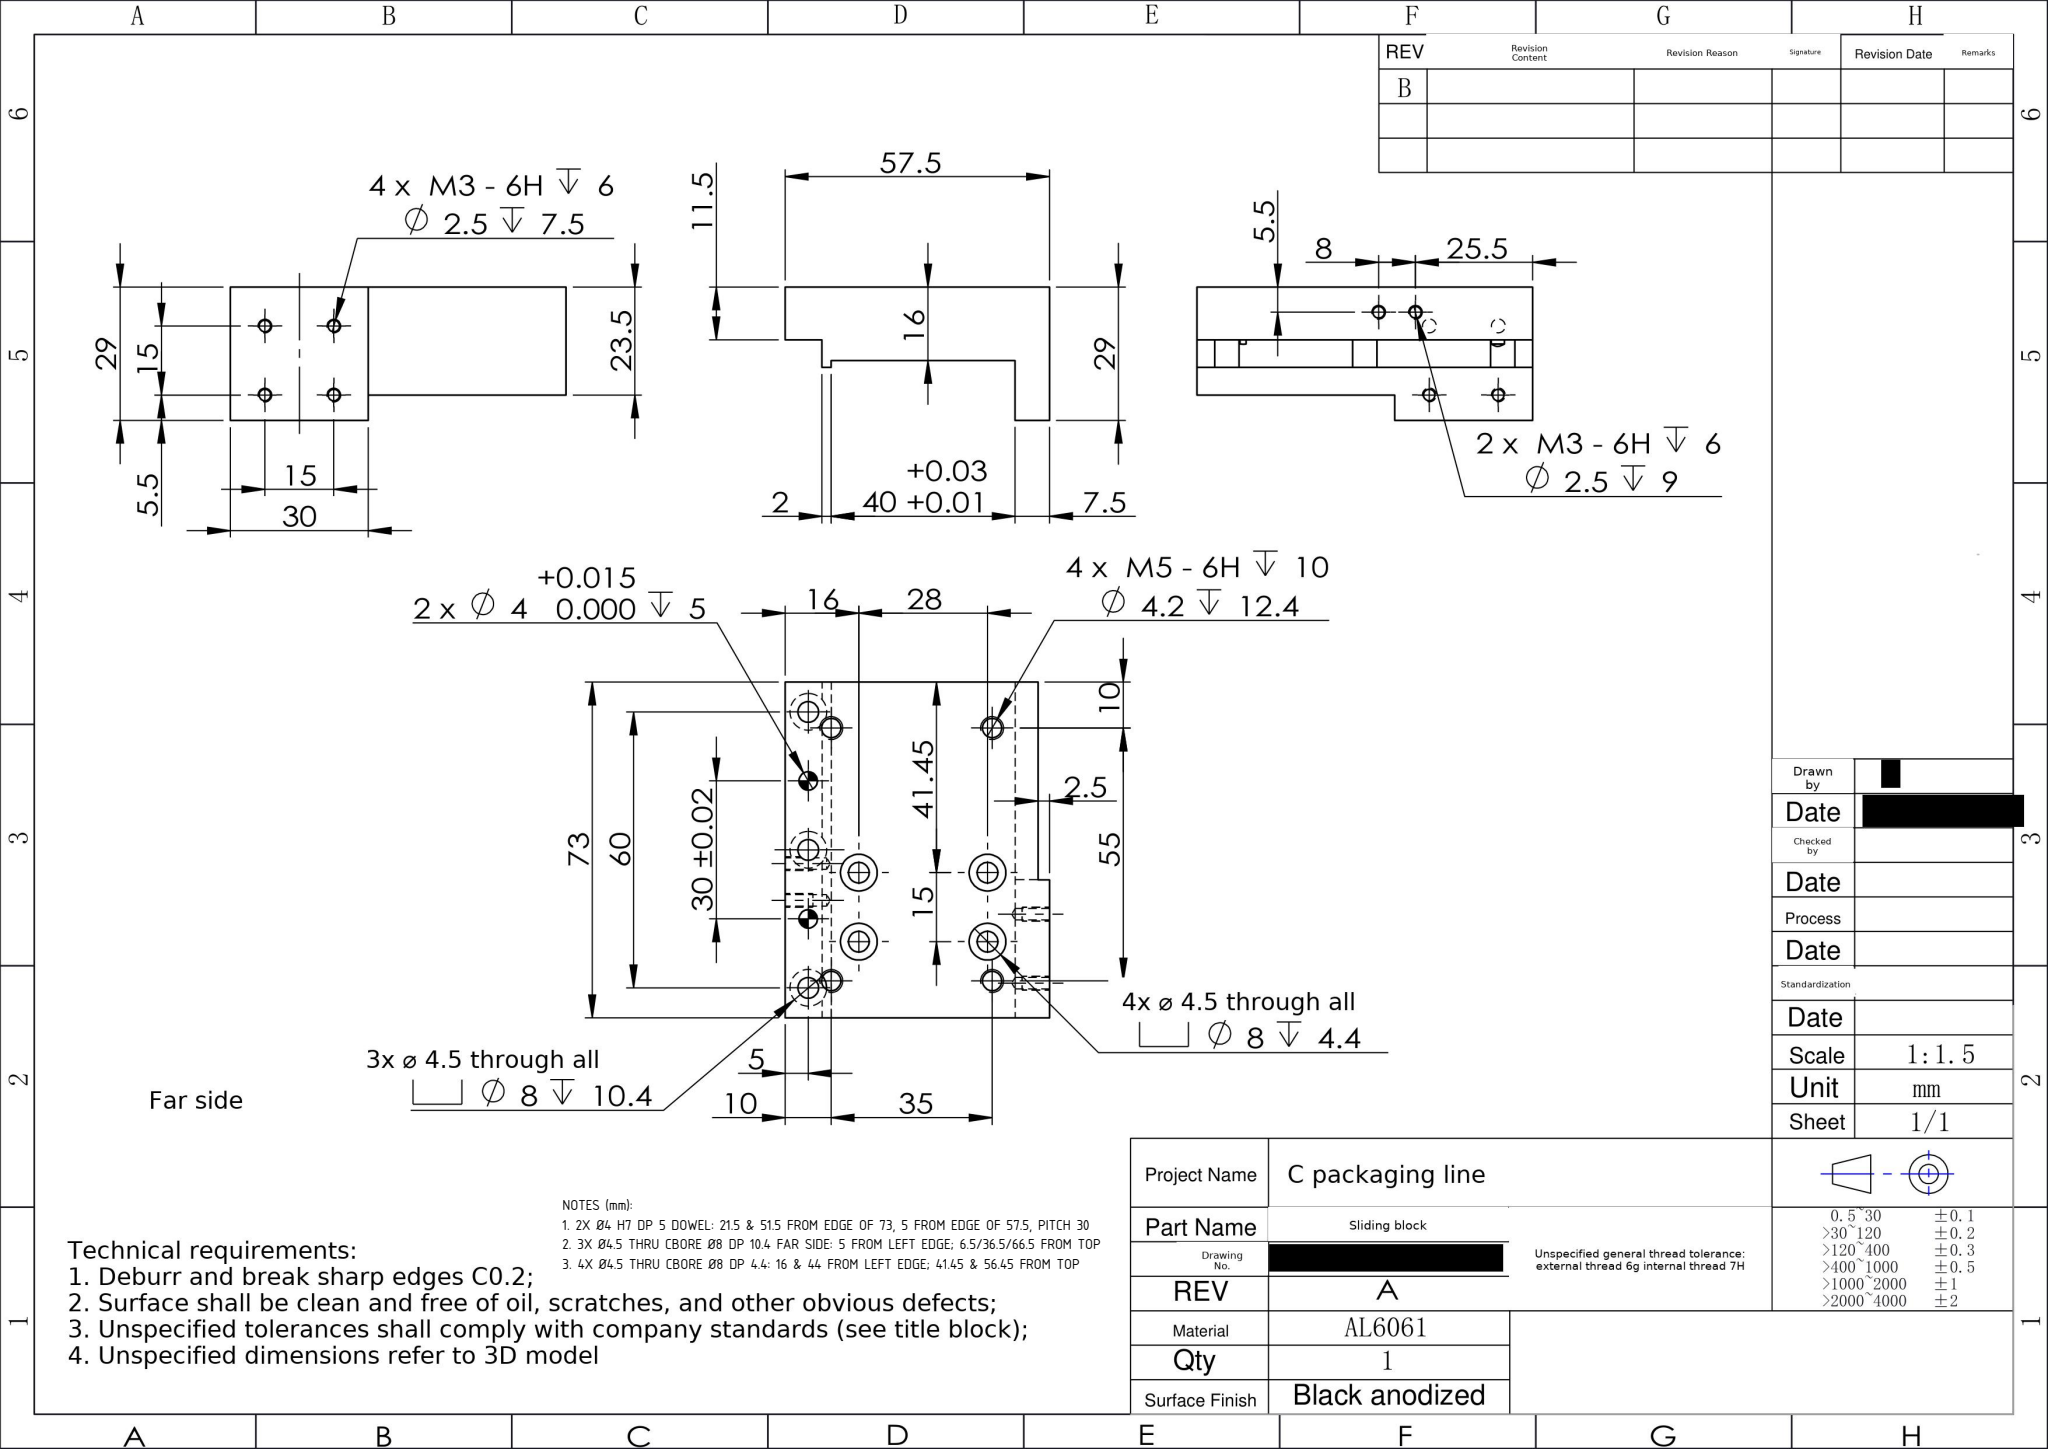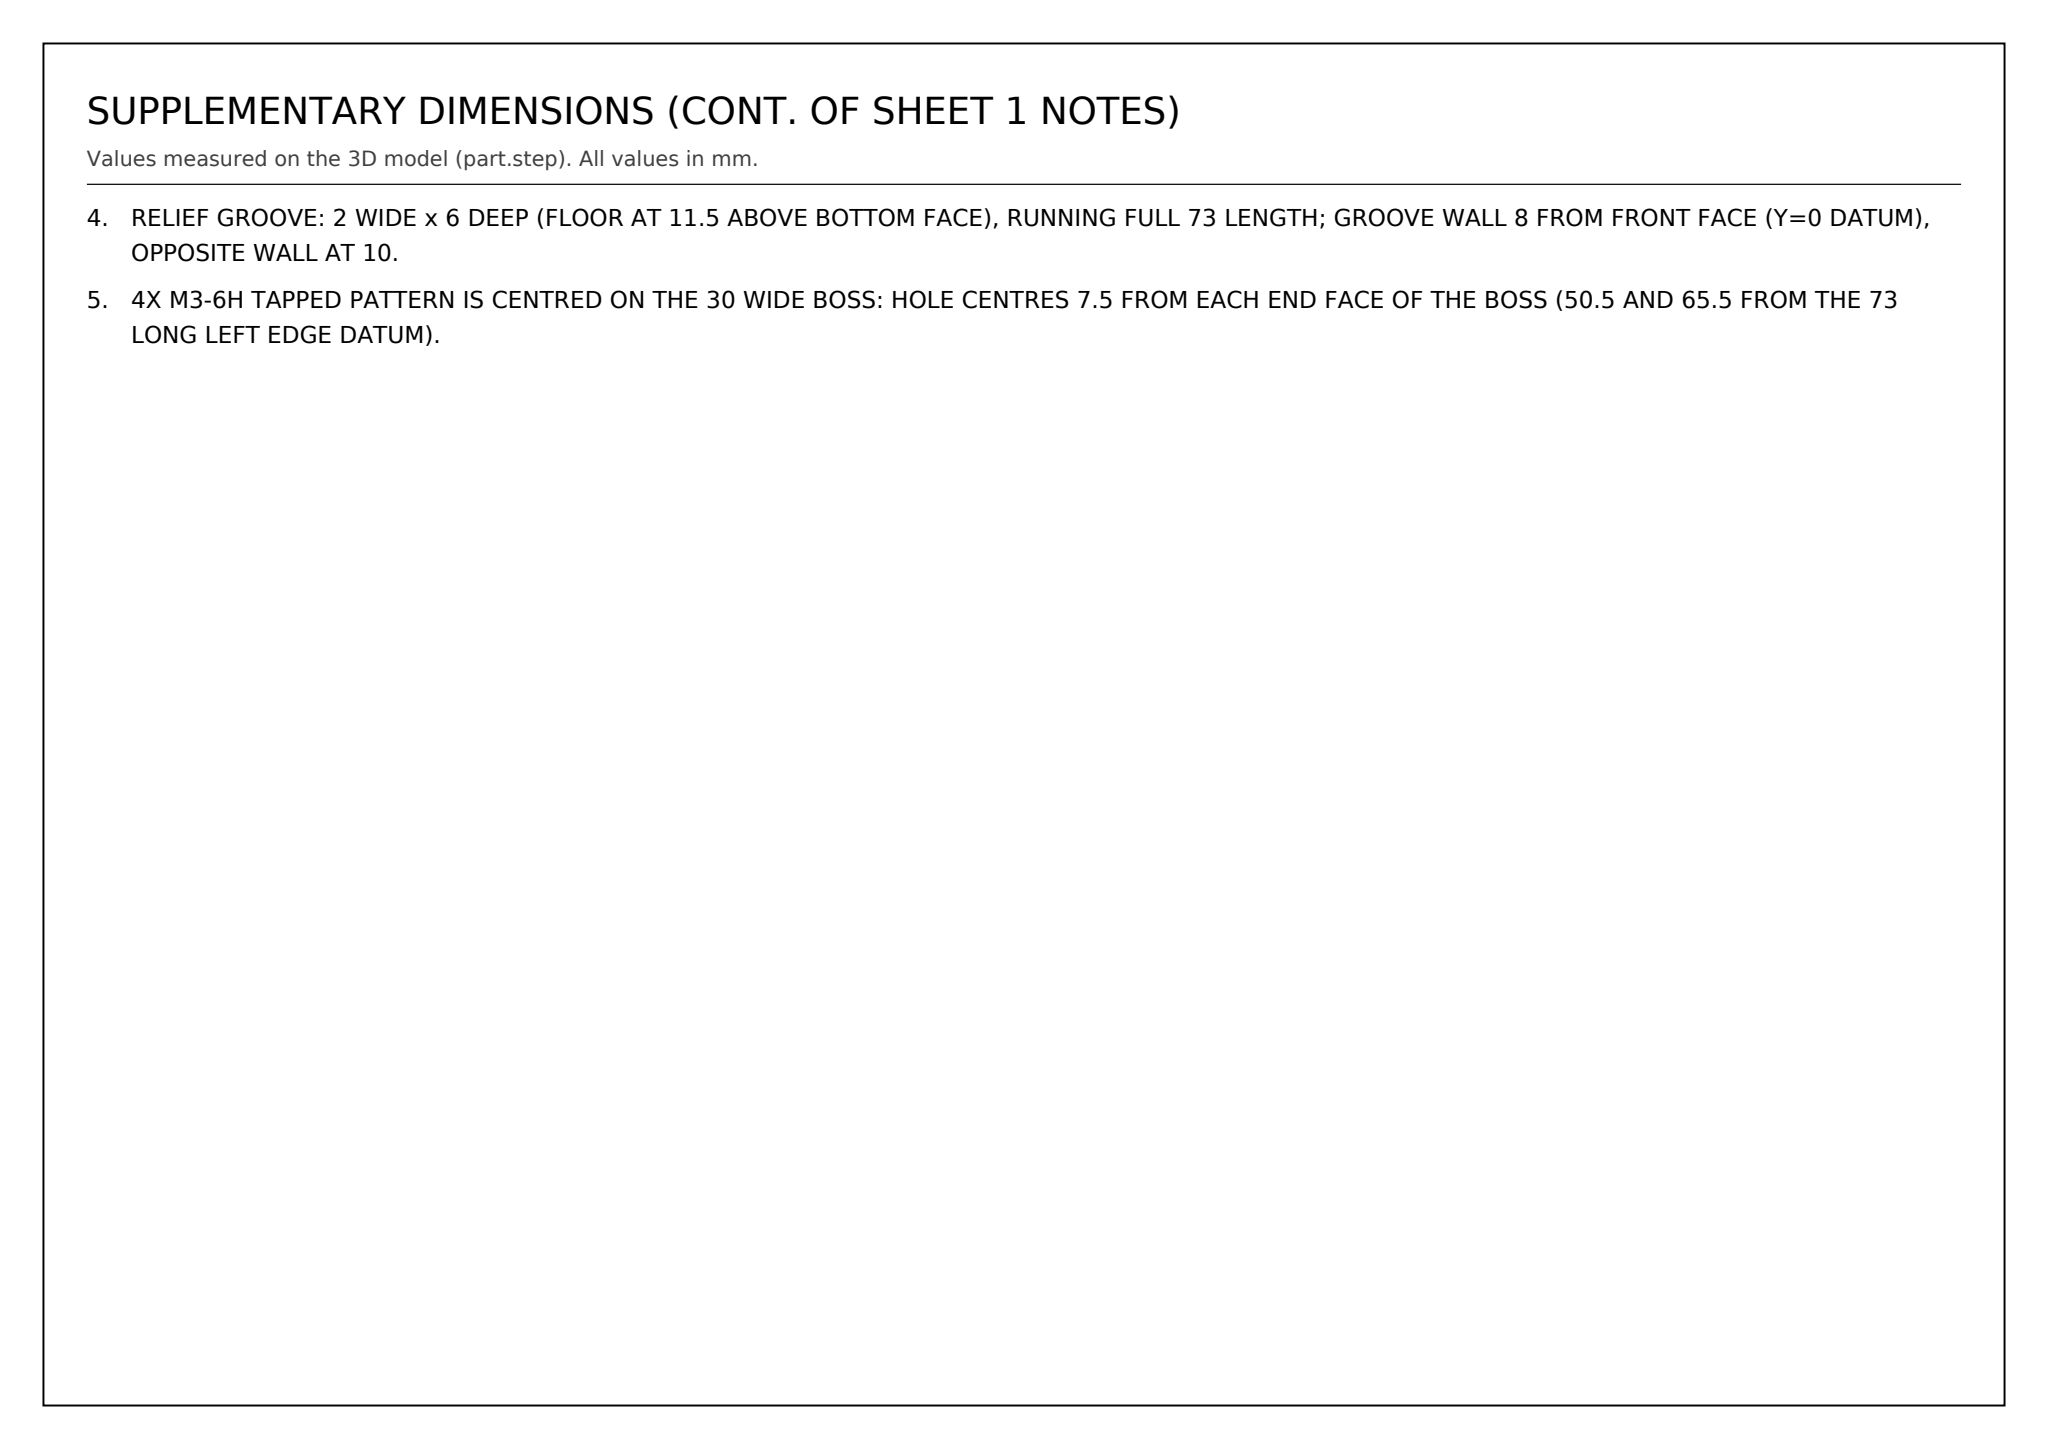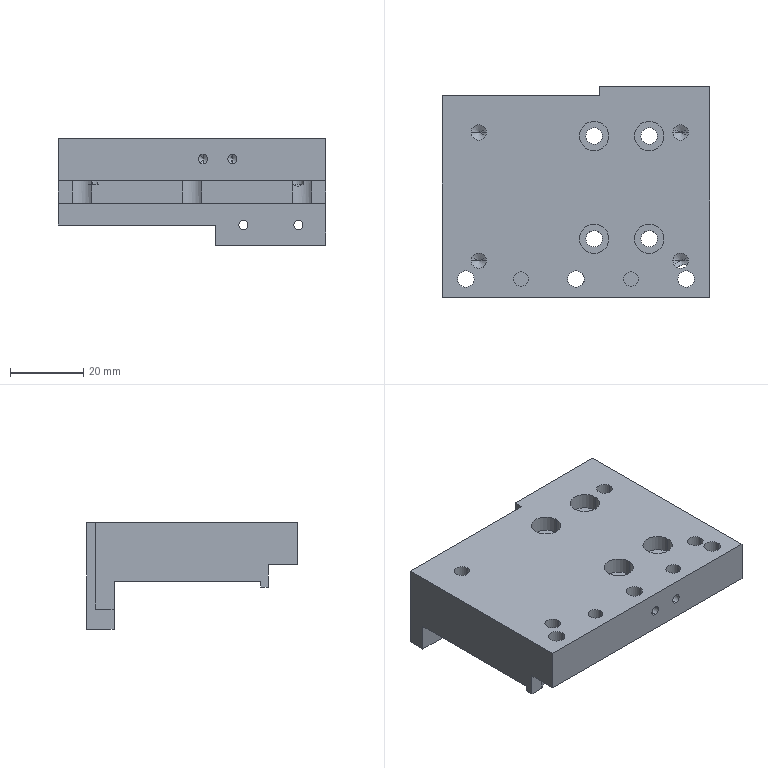Part | SolidWorks | mm | 1 solid | 95 faces | box 73 x 57.5 x 29 mm | volume 63813 mm3 | cylinder 52 | plane 27 | cone 16 | commonest cylinder face diameters 8 x14 4.5 x14 2.5 x12 4.2 x8 4 x4
Drawing notes:
2X Ø4 H7 DP 5 DOWEL: 21.5 & 51.5 FROM EDGE OF 73, 5 FROM EDGE OF 57.5, PITCH 30 | from the solid: Ø4 z-axis holes at (21.5,5.0) & (51.5,5.0), L=5; bbox 73x57.5x29; pitch 30
3X Ø4.5 THRU CBORE Ø8 DP 10.4 FAR SIDE: 5 FROM LEFT EDGE; 6.5/36.5/66.5 FROM TOP | from the solid: Ø4.5 thru holes at (6.5,5.0),(36.5,5.0),(66.5,5.0); Ø8 ↧10.4 same axes
4X Ø4.5 THRU CBORE Ø8 DP 4.4: 16 & 44 FROM LEFT EDGE; 41.45 & 56.45 FROM TOP | from the solid: Ø4.5 holes at (41.45,16),(41.45,44),(56.45,16),(56.45,44); Ø8 ↧4.4
RELIEF GROOVE: 2 WIDE x 6 DEEP (FLOOR AT 11.5 ABOVE BOTTOM FACE), RUNNING FULL 73 LENGTH; GROOVE WALL 8 FROM FRONT FACE (Y=0 DATUM), OPPOSITE WALL AT 10. | from the solid: axis_planes y=8.0 (z 11.5-17.5) and y=10.0 (z 11.5-13.0) with z=11.5 floor plane extent x[0,73], y[8,10]
4X M3-6H TAPPED PATTERN IS CENTRED ON THE 30 WIDE BOSS: HOLE CENTRES 7.5 FROM EACH END FACE OF THE BOSS (50.5 AND 65.5 FROM THE 73 LONG LEFT EDGE DATUM). | from the solid: cylinders dia 2.5 axis y at x=50.5 and x=65.5 (z=20.5 and 5.5), boss faces at x=43.0 and x=73.0
build123d program:
from build123d import *

# Parameters (mm, degrees)
SKETCH1_W                                       = 73
SKETCH1_H                                       = 55
BOSS_EXTRUDE1_DEPTH                             = 11.75
SKETCH2_W                                       = 7.5
SKETCH2_H                                       = 40
CUT_EXTRUDE1_DEPTH                              = 79.888
SKETCH3_W                                       = 10.373
SKETCH3_H                                       = 18.333
CUT_EXTRUDE2_DEPTH                              = 79.888
SKETCH4_W                                       = 30
SKETCH4_H                                       = 23.5
BOSS_EXTRUDE2_DEPTH                             = 4.5
M4_HEX_SOCKET_HEAD_CAP_SCREW_CBORE1_D           = 4.5
M4_HEX_SOCKET_HEAD_CAP_SCREW_CBORE1_DEPTH       = 23.5
M4_HEX_SOCKET_HEAD_CAP_SCREW_CBORE1_CBORE_D     = 8
M4_HEX_SOCKET_HEAD_CAP_SCREW_CBORE1_CBORE_DEPTH = 4.4
M4_HEX_SOCKET_HEAD_CAP_SCREW_CBORE2_D           = 4.5
M4_HEX_SOCKET_HEAD_CAP_SCREW_CBORE2_CBORE_D     = 8
M4_HEX_SOCKET_HEAD_CAP_SCREW_CBORE2_CBORE_DEPTH = 10.4
F_4_0_MM_DOWEL_PIN_HOLE1_D                      = 4
F_4_0_MM_DOWEL_PIN_HOLE1_DEPTH                  = 5
M5_TAPPED_HOLE1_D                               = 4.2
M5_TAPPED_HOLE1_DEPTH                           = 12.4
M5_TAPPED_HOLE1_TIP                             = 1.262
M3_TAPPED_HOLE1_D                               = 2.5
M3_TAPPED_HOLE1_DEPTH                           = 9
M3_TAPPED_HOLE1_TIP                             = 0.7511
SKETCH18_W                                      = 30
SKETCH18_H                                      = 9.5
BOSS_EXTRUDE3_DEPTH                             = 5.5
SKETCH19_W                                      = 30
SKETCH19_H                                      = 29
CUT_EXTRUDE3_DEPTH                              = 2
M3_TAPPED_HOLE2_D                               = 2.5
M3_TAPPED_HOLE2_DEPTH                           = 7.5
M3_TAPPED_HOLE2_TIP                             = 0.7511
SKETCH22_W                                      = 6
SKETCH22_H                                      = 8
CUT_EXTRUDE4_DEPTH                              = 81.787


with BuildPart() as part:
    # Sketch1 → Boss-Extrude1 (new, symmetric)
    with BuildSketch(Plane.XY):
        Rectangle(SKETCH1_W, SKETCH1_H)
    extrude(amount=BOSS_EXTRUDE1_DEPTH, both=True)

    # Sketch2 → Cut-Extrude1 (cut, through all)
    with BuildSketch(Plane(origin=(36.5, 0, 0), x_dir=(0, 0, -1), z_dir=(1, 0, 0))):
        with Locations((8, 2.5)):
            Rectangle(SKETCH2_W, SKETCH2_H)
    extrude(amount=-CUT_EXTRUDE1_DEPTH, mode=Mode.SUBTRACT)

    # Sketch3 → Cut-Extrude2 (cut, through all)
    with BuildSketch(Plane(origin=(36.5, 0, 0), x_dir=(0, 0, -1), z_dir=(1, 0, 0))):
        with Locations((10.936, -24.062)):
            Rectangle(SKETCH3_W, SKETCH3_H)
    extrude(amount=-CUT_EXTRUDE2_DEPTH, mode=Mode.SUBTRACT)

    # Sketch4 → Boss-Extrude2 (add)
    with BuildSketch(Plane(origin=(0, 27.5, 0), x_dir=(1, 0, 0), z_dir=(0, 1, 0))):
        with Locations((21.5, 0)):
            Rectangle(SKETCH4_W, SKETCH4_H)
    extrude(amount=BOSS_EXTRUDE2_DEPTH)

    # M4 Hex Socket Head Cap Screw CBORE1
    with Locations(Plane.XY.offset(11.75)):
        with Locations((4.95, 16.5), (4.95, -11.5), (19.95, -11.5), (19.95, 16.5)):
            CounterBoreHole(M4_HEX_SOCKET_HEAD_CAP_SCREW_CBORE1_D / 2, M4_HEX_SOCKET_HEAD_CAP_SCREW_CBORE1_CBORE_D / 2, M4_HEX_SOCKET_HEAD_CAP_SCREW_CBORE1_CBORE_DEPTH, depth=M4_HEX_SOCKET_HEAD_CAP_SCREW_CBORE1_DEPTH)

    # M4 Hex Socket Head Cap Screw CBORE2 (through all)
    with Locations(Plane(origin=(0, 0, -5.75), x_dir=(-1, 0, 0), z_dir=(0, 0, -1))):
        with Locations((30, -22.5), (0, -22.5), (-30, -22.5)):
            CounterBoreHole(M4_HEX_SOCKET_HEAD_CAP_SCREW_CBORE2_D / 2, M4_HEX_SOCKET_HEAD_CAP_SCREW_CBORE2_CBORE_D / 2, M4_HEX_SOCKET_HEAD_CAP_SCREW_CBORE2_CBORE_DEPTH)

    # 4.0 mm Dowel Pin Hole1
    with Locations(Plane.XY.offset(11.75)):
        with Locations((15, -22.5), (-15, -22.5)):
            Hole(F_4_0_MM_DOWEL_PIN_HOLE1_D / 2, depth=F_4_0_MM_DOWEL_PIN_HOLE1_DEPTH)

    # M5 Tapped Hole1
    with Locations(Plane.XY.offset(11.75)):
        with Locations((28.5, 17.5), (28.5, -17.5), (-26.5, 17.5), (-26.5, -17.5)):
            Hole(M5_TAPPED_HOLE1_D / 2, depth=M5_TAPPED_HOLE1_DEPTH)
            with Locations((0, 0, -(M5_TAPPED_HOLE1_DEPTH + M5_TAPPED_HOLE1_TIP / 2))):  # 118° drill point
                Cone(0, M5_TAPPED_HOLE1_D / 2, M5_TAPPED_HOLE1_TIP, mode=Mode.SUBTRACT)

    # M3 Tapped Hole1
    with Locations(Plane(origin=(0, -27.5, 0), x_dir=(-1, 0, 0), z_dir=(0, -1, 0))):
        with Locations((-11, -6.25), (-3, -6.25)):
            Hole(M3_TAPPED_HOLE1_D / 2, depth=M3_TAPPED_HOLE1_DEPTH)
            with Locations((0, 0, -(M3_TAPPED_HOLE1_DEPTH + M3_TAPPED_HOLE1_TIP / 2))):  # 118° drill point
                Cone(0, M3_TAPPED_HOLE1_D / 2, M3_TAPPED_HOLE1_TIP, mode=Mode.SUBTRACT)

    # Sketch18 → Boss-Extrude3 (add)
    with BuildSketch(Plane(origin=(0, 0, -11.75), x_dir=(-1, 0, 0), z_dir=(0, 0, -1))):
        with Locations((-21.5, 27.25)):
            Rectangle(SKETCH18_W, SKETCH18_H)
    extrude(amount=BOSS_EXTRUDE3_DEPTH)

    # Sketch19 → Cut-Extrude3 (cut)
    with BuildSketch(Plane(origin=(0, 32, 0), x_dir=(1, 0, 0), z_dir=(0, 1, 0))):
        with Locations((21.5, 2.75)):
            Rectangle(SKETCH19_W, SKETCH19_H)
    extrude(amount=-CUT_EXTRUDE3_DEPTH, mode=Mode.SUBTRACT)

    # M3 Tapped Hole2
    with Locations(Plane(origin=(0, 30, 0), x_dir=(1, 0, 0), z_dir=(0, 1, 0))):
        with Locations((14, 11.75), (29, 11.75), (29, -3.25), (14, -3.25)):
            Hole(M3_TAPPED_HOLE2_D / 2, depth=M3_TAPPED_HOLE2_DEPTH)
            with Locations((0, 0, -(M3_TAPPED_HOLE2_DEPTH + M3_TAPPED_HOLE2_TIP / 2))):  # 118° drill point
                Cone(0, M3_TAPPED_HOLE2_D / 2, M3_TAPPED_HOLE2_TIP, mode=Mode.SUBTRACT)

    # Sketch22 → Cut-Extrude4 (cut, through all)
    with BuildSketch(Plane(origin=(36.5, 0, 0), x_dir=(0, 0, -1), z_dir=(1, 0, 0))):
        with Locations((2.75, -23.5)):
            Rectangle(SKETCH22_W, SKETCH22_H)
    extrude(amount=-CUT_EXTRUDE4_DEPTH, mode=Mode.SUBTRACT)


solid = part.part